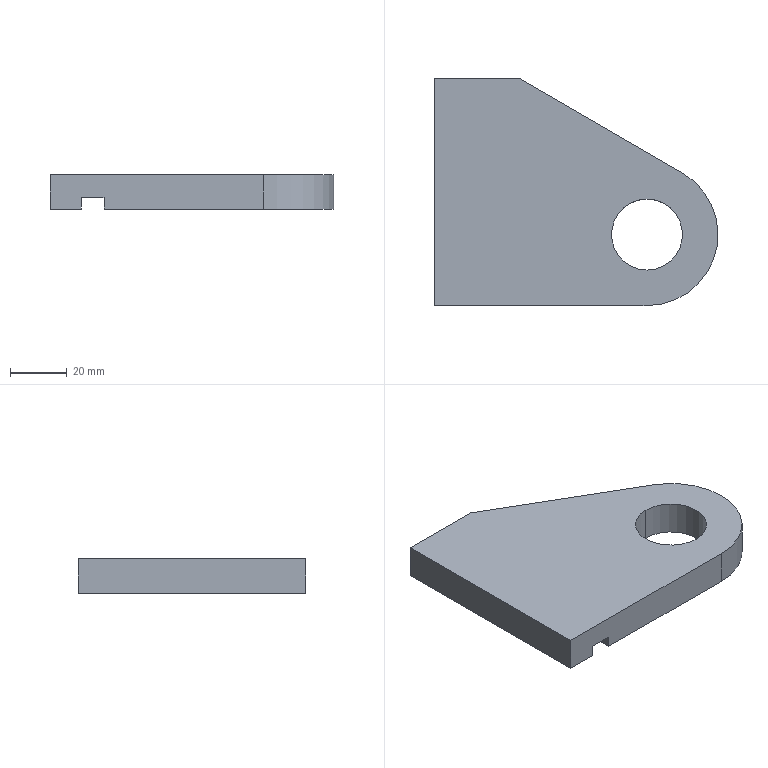Component | SolidWorks | 12AOuterSideWheel-EngravingAndMillingAxis-1_12AOuterSideWheelPlate-1 | 1 solid | 13 faces | box 100 x 80 x 12 mm | volume 68488 mm3 | plane 10 | cylinder 3 | commonest cylinder face diameters 25 x2 50 x1 | material Cr12MoV
build123d program:
from build123d import *

# Parameters (mm, degrees)
SKETCH1_R           = 12.5
BOSS_EXTRUDE1_DEPTH = 12
SKETCH2_W           = 80
SKETCH2_H           = 8
CUT_EXTRUDE1_DEPTH  = 4


with BuildPart() as part:
    # Sketch1 → Boss-Extrude1 (new body)
    with BuildSketch(Plane.XY):
        with BuildLine():
            Line((0, 0), (80, 0))
            Line((80, 0), (80, 30))
            Line((80, 30), (46.626, 87.543))
            ThreePointArc((46.626, 87.543), (18.506, 99.142), (0, 75))
            Line((0, 75), (0, 0))
        make_face()
        with Locations((25, 75)):
            Circle(SKETCH1_R, mode=Mode.SUBTRACT)
    extrude(amount=BOSS_EXTRUDE1_DEPTH)

    # Sketch2 → Cut-Extrude1 (cut)
    with BuildSketch(Plane.XY.offset(12)):
        with Locations((40, 15)):
            Rectangle(SKETCH2_W, SKETCH2_H)
    extrude(amount=-CUT_EXTRUDE1_DEPTH, mode=Mode.SUBTRACT)


solid = part.part

# Placed as in the assembly
solid = solid.moved(Location((196.598, 111.538, 72.25), (180, 0, -90)))
STEP:
#1=COLOUR_RGB('',0.7922,0.8196,0.9333);
#2=FILL_AREA_STYLE_COLOUR('',#1);
#3=FILL_AREA_STYLE('',(#2));
#4=SURFACE_STYLE_FILL_AREA(#3);
#5=SURFACE_SIDE_STYLE('',(#4));
#6=SURFACE_STYLE_USAGE(.BOTH.,#5);
#7=PRESENTATION_STYLE_ASSIGNMENT((#6));
#8=CARTESIAN_POINT('',(10.693,4.883,2.372));
#9=VERTEX_POINT('',#8);
#10=CARTESIAN_POINT('',(10.693,5.868,2.372));
#11=VERTEX_POINT('',#10);
#12=CARTESIAN_POINT('',(10.693,5.376,2.372));
#13=DIRECTION('',(0.,0.,-1.));
#14=DIRECTION('',(0.,1.,0.));
#15=AXIS2_PLACEMENT_3D('',#12,#13,#14);
#16=CIRCLE('',#15,0.4921);
#17=EDGE_CURVE('',#9,#11,#16,.T.);
#18=ORIENTED_EDGE('',*,*,#17,.T.);
#19=CARTESIAN_POINT('',(10.693,5.868,2.844));
#20=VERTEX_POINT('',#19);
#21=CARTESIAN_POINT('',(10.693,5.868,2.372));
#22=DIRECTION('',(0.,0.,1.));
#23=VECTOR('',#22,39.37);
#24=LINE('',#21,#23);
#25=EDGE_CURVE('',#11,#20,#24,.T.);
#26=ORIENTED_EDGE('',*,*,#25,.T.);
#27=CARTESIAN_POINT('',(10.693,4.883,2.844));
#28=VERTEX_POINT('',#27);
#29=CARTESIAN_POINT('',(10.693,5.376,2.844));
#30=DIRECTION('',(0.,0.,-1.));
#31=DIRECTION('',(0.,1.,0.));
#32=AXIS2_PLACEMENT_3D('',#29,#30,#31);
#33=CIRCLE('',#32,0.4921);
#34=EDGE_CURVE('',#28,#20,#33,.T.);
#35=ORIENTED_EDGE('',*,*,#34,.F.);
#36=CARTESIAN_POINT('',(10.693,4.883,2.372));
#37=DIRECTION('',(0.,0.,1.));
#38=VECTOR('',#37,39.37);
#39=LINE('',#36,#38);
#40=EDGE_CURVE('',#9,#28,#39,.T.);
#41=ORIENTED_EDGE('',*,*,#40,.F.);
#42=EDGE_LOOP('',(#18,#26,#35,#41));
#43=FACE_OUTER_BOUND('',#42,.T.);
#44=CARTESIAN_POINT('',(10.693,5.376,2.372));
#45=DIRECTION('',(0.,0.,1.));
#46=DIRECTION('',(0.,-1.,0.));
#47=AXIS2_PLACEMENT_3D('',#44,#45,#46);
#48=CYLINDRICAL_SURFACE('',#47,0.4921);
#49=ADVANCED_FACE('',(#43),#48,.F.);
#50=CARTESIAN_POINT('',(8.488,7.541,2.372));
#51=VERTEX_POINT('',#50);
#52=CARTESIAN_POINT('',(8.488,4.391,2.372));
#53=VERTEX_POINT('',#52);
#54=CARTESIAN_POINT('',(8.488,4.391,2.372));
#55=DIRECTION('',(-0.,-1.,0.));
#56=VECTOR('',#55,39.37);
#57=LINE('',#54,#56);
#58=EDGE_CURVE('',#51,#53,#57,.T.);
#59=ORIENTED_EDGE('',*,*,#58,.F.);
#60=CARTESIAN_POINT('',(8.921,7.541,2.372));
#61=VERTEX_POINT('',#60);
#62=CARTESIAN_POINT('',(7.74,7.541,2.372));
#63=DIRECTION('',(1.,0.,0.));
#64=VECTOR('',#63,39.37);
#65=LINE('',#62,#64);
#66=EDGE_CURVE('',#51,#61,#65,.T.);
#67=ORIENTED_EDGE('',*,*,#66,.T.);
#68=CARTESIAN_POINT('',(11.187,6.227,2.372));
#69=VERTEX_POINT('',#68);
#70=CARTESIAN_POINT('',(8.921,7.541,2.372));
#71=DIRECTION('',(0.865,-0.5017,0.));
#72=VECTOR('',#71,39.37);
#73=LINE('',#70,#72);
#74=EDGE_CURVE('',#61,#69,#73,.T.);
#75=ORIENTED_EDGE('',*,*,#74,.T.);
#76=CARTESIAN_POINT('',(10.693,4.391,2.372));
#77=VERTEX_POINT('',#76);
#78=CARTESIAN_POINT('',(10.693,5.376,2.372));
#79=DIRECTION('',(0.,0.,-1.));
#80=DIRECTION('',(0.,1.,0.));
#81=AXIS2_PLACEMENT_3D('',#78,#79,#80);
#82=CIRCLE('',#81,0.9843);
#83=EDGE_CURVE('',#69,#77,#82,.T.);
#84=ORIENTED_EDGE('',*,*,#83,.T.);
#85=CARTESIAN_POINT('',(7.74,4.391,2.372));
#86=DIRECTION('',(-1.,0.,0.));
#87=VECTOR('',#86,39.37);
#88=LINE('',#85,#87);
#89=EDGE_CURVE('',#77,#53,#88,.T.);
#90=ORIENTED_EDGE('',*,*,#89,.T.);
#91=EDGE_LOOP('',(#59,#67,#75,#84,#90));
#92=FACE_OUTER_BOUND('',#91,.T.);
#93=ORIENTED_EDGE('',*,*,#17,.F.);
#94=CARTESIAN_POINT('',(10.693,5.376,2.372));
#95=DIRECTION('',(0.,0.,-1.));
#96=DIRECTION('',(0.,1.,0.));
#97=AXIS2_PLACEMENT_3D('',#94,#95,#96);
#98=CIRCLE('',#97,0.4921);
#99=EDGE_CURVE('',#11,#9,#98,.T.);
#100=ORIENTED_EDGE('',*,*,#99,.F.);
#101=EDGE_LOOP('',(#93,#100));
#102=FACE_BOUND('',#101,.T.);
#103=CARTESIAN_POINT('',(10.693,5.376,2.372));
#104=DIRECTION('',(0.,0.,-1.));
#105=DIRECTION('',(0.,1.,0.));
#106=AXIS2_PLACEMENT_3D('',#103,#104,#105);
#107=PLANE('',#106);
#108=ADVANCED_FACE('',(#92,#102),#107,.T.);
#109=CARTESIAN_POINT('',(8.173,4.391,2.372));
#110=VERTEX_POINT('',#109);
#111=CARTESIAN_POINT('',(8.173,7.541,2.372));
#112=VERTEX_POINT('',#111);
#113=CARTESIAN_POINT('',(8.173,4.391,2.372));
#114=DIRECTION('',(0.,1.,0.));
#115=VECTOR('',#114,39.37);
#116=LINE('',#113,#115);
#117=EDGE_CURVE('',#110,#112,#116,.T.);
#118=ORIENTED_EDGE('',*,*,#117,.F.);
#119=CARTESIAN_POINT('',(7.74,4.391,2.372));
#120=VERTEX_POINT('',#119);
#121=CARTESIAN_POINT('',(7.74,4.391,2.372));
#122=DIRECTION('',(-1.,0.,0.));
#123=VECTOR('',#122,39.37);
#124=LINE('',#121,#123);
#125=EDGE_CURVE('',#110,#120,#124,.T.);
#126=ORIENTED_EDGE('',*,*,#125,.T.);
#127=CARTESIAN_POINT('',(7.74,7.541,2.372));
#128=VERTEX_POINT('',#127);
#129=CARTESIAN_POINT('',(7.74,4.391,2.372));
#130=DIRECTION('',(0.,1.,0.));
#131=VECTOR('',#130,39.37);
#132=LINE('',#129,#131);
#133=EDGE_CURVE('',#120,#128,#132,.T.);
#134=ORIENTED_EDGE('',*,*,#133,.T.);
#135=CARTESIAN_POINT('',(7.74,7.541,2.372));
#136=DIRECTION('',(1.,0.,0.));
#137=VECTOR('',#136,39.37);
#138=LINE('',#135,#137);
#139=EDGE_CURVE('',#128,#112,#138,.T.);
#140=ORIENTED_EDGE('',*,*,#139,.T.);
#141=EDGE_LOOP('',(#118,#126,#134,#140));
#142=FACE_OUTER_BOUND('',#141,.T.);
#143=CARTESIAN_POINT('',(10.693,5.376,2.372));
#144=DIRECTION('',(0.,0.,-1.));
#145=DIRECTION('',(0.,1.,0.));
#146=AXIS2_PLACEMENT_3D('',#143,#144,#145);
#147=PLANE('',#146);
#148=ADVANCED_FACE('',(#142),#147,.T.);
#149=CARTESIAN_POINT('',(10.693,4.391,2.844));
#150=VERTEX_POINT('',#149);
#151=CARTESIAN_POINT('',(7.74,4.391,2.844));
#152=VERTEX_POINT('',#151);
#153=CARTESIAN_POINT('',(7.74,4.391,2.844));
#154=DIRECTION('',(-1.,0.,0.));
#155=VECTOR('',#154,39.37);
#156=LINE('',#153,#155);
#157=EDGE_CURVE('',#150,#152,#156,.T.);
#158=ORIENTED_EDGE('',*,*,#157,.F.);
#159=CARTESIAN_POINT('',(11.187,6.227,2.844));
#160=VERTEX_POINT('',#159);
#161=CARTESIAN_POINT('',(10.693,5.376,2.844));
#162=DIRECTION('',(0.,0.,-1.));
#163=DIRECTION('',(0.,1.,0.));
#164=AXIS2_PLACEMENT_3D('',#161,#162,#163);
#165=CIRCLE('',#164,0.9843);
#166=EDGE_CURVE('',#160,#150,#165,.T.);
#167=ORIENTED_EDGE('',*,*,#166,.F.);
#168=CARTESIAN_POINT('',(8.921,7.541,2.844));
#169=VERTEX_POINT('',#168);
#170=CARTESIAN_POINT('',(8.921,7.541,2.844));
#171=DIRECTION('',(0.865,-0.5017,0.));
#172=VECTOR('',#171,39.37);
#173=LINE('',#170,#172);
#174=EDGE_CURVE('',#169,#160,#173,.T.);
#175=ORIENTED_EDGE('',*,*,#174,.F.);
#176=CARTESIAN_POINT('',(7.74,7.541,2.844));
#177=VERTEX_POINT('',#176);
#178=CARTESIAN_POINT('',(7.74,7.541,2.844));
#179=DIRECTION('',(1.,0.,0.));
#180=VECTOR('',#179,39.37);
#181=LINE('',#178,#180);
#182=EDGE_CURVE('',#177,#169,#181,.T.);
#183=ORIENTED_EDGE('',*,*,#182,.F.);
#184=CARTESIAN_POINT('',(7.74,4.391,2.844));
#185=DIRECTION('',(0.,1.,0.));
#186=VECTOR('',#185,39.37);
#187=LINE('',#184,#186);
#188=EDGE_CURVE('',#152,#177,#187,.T.);
#189=ORIENTED_EDGE('',*,*,#188,.F.);
#190=EDGE_LOOP('',(#158,#167,#175,#183,#189));
#191=FACE_OUTER_BOUND('',#190,.T.);
#192=ORIENTED_EDGE('',*,*,#34,.T.);
#193=CARTESIAN_POINT('',(10.693,5.376,2.844));
#194=DIRECTION('',(0.,0.,-1.));
#195=DIRECTION('',(0.,1.,0.));
#196=AXIS2_PLACEMENT_3D('',#193,#194,#195);
#197=CIRCLE('',#196,0.4921);
#198=EDGE_CURVE('',#20,#28,#197,.T.);
#199=ORIENTED_EDGE('',*,*,#198,.T.);
#200=EDGE_LOOP('',(#192,#199));
#201=FACE_BOUND('',#200,.T.);
#202=CARTESIAN_POINT('',(10.693,5.376,2.844));
#203=DIRECTION('',(0.,0.,-1.));
#204=DIRECTION('',(0.,1.,0.));
#205=AXIS2_PLACEMENT_3D('',#202,#203,#204);
#206=PLANE('',#205);
#207=ADVANCED_FACE('',(#191,#201),#206,.F.);
#208=CARTESIAN_POINT('',(8.488,4.391,2.53));
#209=VERTEX_POINT('',#208);
#210=CARTESIAN_POINT('',(8.173,4.391,2.53));
#211=VERTEX_POINT('',#210);
#212=CARTESIAN_POINT('',(8.173,4.391,2.53));
#213=DIRECTION('',(-1.,0.,0.));
#214=VECTOR('',#213,39.37);
#215=LINE('',#212,#214);
#216=EDGE_CURVE('',#209,#211,#215,.T.);
#217=ORIENTED_EDGE('',*,*,#216,.F.);
#218=CARTESIAN_POINT('',(8.488,4.391,2.53));
#219=DIRECTION('',(0.,0.,-1.));
#220=VECTOR('',#219,39.37);
#221=LINE('',#218,#220);
#222=EDGE_CURVE('',#209,#53,#221,.T.);
#223=ORIENTED_EDGE('',*,*,#222,.T.);
#224=ORIENTED_EDGE('',*,*,#89,.F.);
#225=CARTESIAN_POINT('',(10.693,4.391,2.372));
#226=DIRECTION('',(0.,0.,1.));
#227=VECTOR('',#226,39.37);
#228=LINE('',#225,#227);
#229=EDGE_CURVE('',#77,#150,#228,.T.);
#230=ORIENTED_EDGE('',*,*,#229,.T.);
#231=ORIENTED_EDGE('',*,*,#157,.T.);
#232=CARTESIAN_POINT('',(7.74,4.391,2.372));
#233=DIRECTION('',(0.,0.,1.));
#234=VECTOR('',#233,39.37);
#235=LINE('',#232,#234);
#236=EDGE_CURVE('',#120,#152,#235,.T.);
#237=ORIENTED_EDGE('',*,*,#236,.F.);
#238=ORIENTED_EDGE('',*,*,#125,.F.);
#239=CARTESIAN_POINT('',(8.173,4.391,2.53));
#240=DIRECTION('',(0.,0.,-1.));
#241=VECTOR('',#240,39.37);
#242=LINE('',#239,#241);
#243=EDGE_CURVE('',#211,#110,#242,.T.);
#244=ORIENTED_EDGE('',*,*,#243,.F.);
#245=EDGE_LOOP('',(#217,#223,#224,#230,#231,#237,#238,#244));
#246=FACE_OUTER_BOUND('',#245,.T.);
#247=CARTESIAN_POINT('',(7.74,4.391,2.372));
#248=DIRECTION('',(0.,1.,0.));
#249=DIRECTION('',(0.,0.,1.));
#250=AXIS2_PLACEMENT_3D('',#247,#248,#249);
#251=PLANE('',#250);
#252=ADVANCED_FACE('',(#246),#251,.F.);
#253=ORIENTED_EDGE('',*,*,#188,.T.);
#254=CARTESIAN_POINT('',(7.74,7.541,2.372));
#255=DIRECTION('',(0.,0.,1.));
#256=VECTOR('',#255,39.37);
#257=LINE('',#254,#256);
#258=EDGE_CURVE('',#128,#177,#257,.T.);
#259=ORIENTED_EDGE('',*,*,#258,.F.);
#260=ORIENTED_EDGE('',*,*,#133,.F.);
#261=ORIENTED_EDGE('',*,*,#236,.T.);
#262=EDGE_LOOP('',(#253,#259,#260,#261));
#263=FACE_OUTER_BOUND('',#262,.T.);
#264=CARTESIAN_POINT('',(7.74,4.391,2.372));
#265=DIRECTION('',(1.,0.,0.));
#266=DIRECTION('',(0.,0.,-1.));
#267=AXIS2_PLACEMENT_3D('',#264,#265,#266);
#268=PLANE('',#267);
#269=ADVANCED_FACE('',(#263),#268,.F.);
#270=ORIENTED_EDGE('',*,*,#66,.F.);
#271=CARTESIAN_POINT('',(8.488,7.541,2.53));
#272=VERTEX_POINT('',#271);
#273=CARTESIAN_POINT('',(8.488,7.541,2.53));
#274=DIRECTION('',(0.,0.,-1.));
#275=VECTOR('',#274,39.37);
#276=LINE('',#273,#275);
#277=EDGE_CURVE('',#272,#51,#276,.T.);
#278=ORIENTED_EDGE('',*,*,#277,.F.);
#279=CARTESIAN_POINT('',(8.173,7.541,2.53));
#280=VERTEX_POINT('',#279);
#281=CARTESIAN_POINT('',(8.173,7.541,2.53));
#282=DIRECTION('',(1.,0.,0.));
#283=VECTOR('',#282,39.37);
#284=LINE('',#281,#283);
#285=EDGE_CURVE('',#280,#272,#284,.T.);
#286=ORIENTED_EDGE('',*,*,#285,.F.);
#287=CARTESIAN_POINT('',(8.173,7.541,2.53));
#288=DIRECTION('',(0.,0.,-1.));
#289=VECTOR('',#288,39.37);
#290=LINE('',#287,#289);
#291=EDGE_CURVE('',#280,#112,#290,.T.);
#292=ORIENTED_EDGE('',*,*,#291,.T.);
#293=ORIENTED_EDGE('',*,*,#139,.F.);
#294=ORIENTED_EDGE('',*,*,#258,.T.);
#295=ORIENTED_EDGE('',*,*,#182,.T.);
#296=CARTESIAN_POINT('',(8.921,7.541,2.372));
#297=DIRECTION('',(0.,0.,1.));
#298=VECTOR('',#297,39.37);
#299=LINE('',#296,#298);
#300=EDGE_CURVE('',#61,#169,#299,.T.);
#301=ORIENTED_EDGE('',*,*,#300,.F.);
#302=EDGE_LOOP('',(#270,#278,#286,#292,#293,#294,#295,#301));
#303=FACE_OUTER_BOUND('',#302,.T.);
#304=CARTESIAN_POINT('',(7.74,7.541,2.372));
#305=DIRECTION('',(0.,-1.,0.));
#306=DIRECTION('',(-1.,-0.,0.));
#307=AXIS2_PLACEMENT_3D('',#304,#305,#306);
#308=PLANE('',#307);
#309=ADVANCED_FACE('',(#303),#308,.F.);
#310=ORIENTED_EDGE('',*,*,#174,.T.);
#311=CARTESIAN_POINT('',(11.187,6.227,2.372));
#312=DIRECTION('',(0.,0.,1.));
#313=VECTOR('',#312,39.37);
#314=LINE('',#311,#313);
#315=EDGE_CURVE('',#69,#160,#314,.T.);
#316=ORIENTED_EDGE('',*,*,#315,.F.);
#317=ORIENTED_EDGE('',*,*,#74,.F.);
#318=ORIENTED_EDGE('',*,*,#300,.T.);
#319=EDGE_LOOP('',(#310,#316,#317,#318));
#320=FACE_OUTER_BOUND('',#319,.T.);
#321=CARTESIAN_POINT('',(8.921,7.541,2.372));
#322=DIRECTION('',(-0.5017,-0.865,0.));
#323=DIRECTION('',(-0.865,0.5017,0.));
#324=AXIS2_PLACEMENT_3D('',#321,#322,#323);
#325=PLANE('',#324);
#326=ADVANCED_FACE('',(#320),#325,.F.);
#327=ORIENTED_EDGE('',*,*,#166,.T.);
#328=ORIENTED_EDGE('',*,*,#229,.F.);
#329=ORIENTED_EDGE('',*,*,#83,.F.);
#330=ORIENTED_EDGE('',*,*,#315,.T.);
#331=EDGE_LOOP('',(#327,#328,#329,#330));
#332=FACE_OUTER_BOUND('',#331,.T.);
#333=CARTESIAN_POINT('',(10.693,5.376,2.372));
#334=DIRECTION('',(0.,0.,1.));
#335=DIRECTION('',(0.,-1.,0.));
#336=AXIS2_PLACEMENT_3D('',#333,#334,#335);
#337=CYLINDRICAL_SURFACE('',#336,0.9843);
#338=ADVANCED_FACE('',(#332),#337,.T.);
#339=ORIENTED_EDGE('',*,*,#25,.F.);
#340=ORIENTED_EDGE('',*,*,#99,.T.);
#341=ORIENTED_EDGE('',*,*,#40,.T.);
#342=ORIENTED_EDGE('',*,*,#198,.F.);
#343=EDGE_LOOP('',(#339,#340,#341,#342));
#344=FACE_OUTER_BOUND('',#343,.T.);
#345=CARTESIAN_POINT('',(10.693,5.376,2.372));
#346=DIRECTION('',(0.,0.,1.));
#347=DIRECTION('',(0.,-1.,0.));
#348=AXIS2_PLACEMENT_3D('',#345,#346,#347);
#349=CYLINDRICAL_SURFACE('',#348,0.4921);
#350=ADVANCED_FACE('',(#344),#349,.F.);
#351=ORIENTED_EDGE('',*,*,#58,.T.);
#352=ORIENTED_EDGE('',*,*,#222,.F.);
#353=CARTESIAN_POINT('',(8.488,4.391,2.53));
#354=DIRECTION('',(-0.,-1.,0.));
#355=VECTOR('',#354,39.37);
#356=LINE('',#353,#355);
#357=EDGE_CURVE('',#272,#209,#356,.T.);
#358=ORIENTED_EDGE('',*,*,#357,.F.);
#359=ORIENTED_EDGE('',*,*,#277,.T.);
#360=EDGE_LOOP('',(#351,#352,#358,#359));
#361=FACE_OUTER_BOUND('',#360,.T.);
#362=CARTESIAN_POINT('',(8.488,4.391,2.53));
#363=DIRECTION('',(1.,-0.,0.));
#364=DIRECTION('',(-0.,-1.,0.));
#365=AXIS2_PLACEMENT_3D('',#362,#363,#364);
#366=PLANE('',#365);
#367=ADVANCED_FACE('',(#361),#366,.F.);
#368=ORIENTED_EDGE('',*,*,#117,.T.);
#369=ORIENTED_EDGE('',*,*,#291,.F.);
#370=CARTESIAN_POINT('',(8.173,4.391,2.53));
#371=DIRECTION('',(0.,1.,0.));
#372=VECTOR('',#371,39.37);
#373=LINE('',#370,#372);
#374=EDGE_CURVE('',#211,#280,#373,.T.);
#375=ORIENTED_EDGE('',*,*,#374,.F.);
#376=ORIENTED_EDGE('',*,*,#243,.T.);
#377=EDGE_LOOP('',(#368,#369,#375,#376));
#378=FACE_OUTER_BOUND('',#377,.T.);
#379=CARTESIAN_POINT('',(8.173,4.391,2.53));
#380=DIRECTION('',(-1.,0.,0.));
#381=DIRECTION('',(0.,1.,0.));
#382=AXIS2_PLACEMENT_3D('',#379,#380,#381);
#383=PLANE('',#382);
#384=ADVANCED_FACE('',(#378),#383,.F.);
#385=ORIENTED_EDGE('',*,*,#216,.T.);
#386=ORIENTED_EDGE('',*,*,#374,.T.);
#387=ORIENTED_EDGE('',*,*,#285,.T.);
#388=ORIENTED_EDGE('',*,*,#357,.T.);
#389=EDGE_LOOP('',(#385,#386,#387,#388));
#390=FACE_OUTER_BOUND('',#389,.T.);
#391=CARTESIAN_POINT('',(7.74,4.391,2.53));
#392=DIRECTION('',(0.,0.,1.));
#393=DIRECTION('',(0.,-1.,0.));
#394=AXIS2_PLACEMENT_3D('',#391,#392,#393);
#395=PLANE('',#394);
#396=ADVANCED_FACE('',(#390),#395,.F.);
#397=CLOSED_SHELL('',(#49,#108,#148,#207,#252,#269,#309,#326,#338,#350,#367,#384,#396));
#398=MANIFOLD_SOLID_BREP('',#397);
#399=STYLED_ITEM('',(#7),#398);
#400=PRESENTATION_LAYER_ASSIGNMENT('','',(#399));
#401=CARTESIAN_POINT('',(0.,0.,0.));
#402=DIRECTION('',(0.,0.,1.));
#403=DIRECTION('',(1.,0.,0.));
#404=AXIS2_PLACEMENT_3D('',#401,#402,#403);
#405=(LENGTH_UNIT()NAMED_UNIT(*)SI_UNIT($,.METRE.));
#406=LENGTH_MEASURE_WITH_UNIT(LENGTH_MEASURE(0.0254),#405);
#407=DIMENSIONAL_EXPONENTS(1.,0.,0.,0.,0.,0.,0.);
#408=(CONVERSION_BASED_UNIT('',#406)LENGTH_UNIT()NAMED_UNIT(#407));
#409=UNCERTAINTY_MEASURE_WITH_UNIT(LENGTH_MEASURE(0.00001),#408,'','');
#410=(NAMED_UNIT(*)PLANE_ANGLE_UNIT()SI_UNIT($,.RADIAN.));
#411=(NAMED_UNIT(*)SI_UNIT($,.STERADIAN.)SOLID_ANGLE_UNIT());
#412=(GEOMETRIC_REPRESENTATION_CONTEXT(3)GLOBAL_UNCERTAINTY_ASSIGNED_CONTEXT((#409))GLOBAL_UNIT_ASSIGNED_CONTEXT((#408,#410,#411))REPRESENTATION_CONTEXT('',''));
#413=ADVANCED_BREP_SHAPE_REPRESENTATION('',(#398,#404),#412);
#414=(LENGTH_UNIT()NAMED_UNIT(*)SI_UNIT($,.METRE.));
#415=LENGTH_MEASURE_WITH_UNIT(LENGTH_MEASURE(0.0254),#414);
#416=DIMENSIONAL_EXPONENTS(1.,0.,0.,0.,0.,0.,0.);
#417=(CONVERSION_BASED_UNIT('',#415)LENGTH_UNIT()NAMED_UNIT(#416));
#418=UNCERTAINTY_MEASURE_WITH_UNIT(LENGTH_MEASURE(0.00001),#417,'','');
#419=(NAMED_UNIT(*)PLANE_ANGLE_UNIT()SI_UNIT($,.RADIAN.));
#420=(NAMED_UNIT(*)SI_UNIT($,.STERADIAN.)SOLID_ANGLE_UNIT());
#421=(GEOMETRIC_REPRESENTATION_CONTEXT(3)GLOBAL_UNCERTAINTY_ASSIGNED_CONTEXT((#418))GLOBAL_UNIT_ASSIGNED_CONTEXT((#417,#419,#420))REPRESENTATION_CONTEXT('',''));
#422=MECHANICAL_DESIGN_GEOMETRIC_PRESENTATION_REPRESENTATION('',(#399),#421);